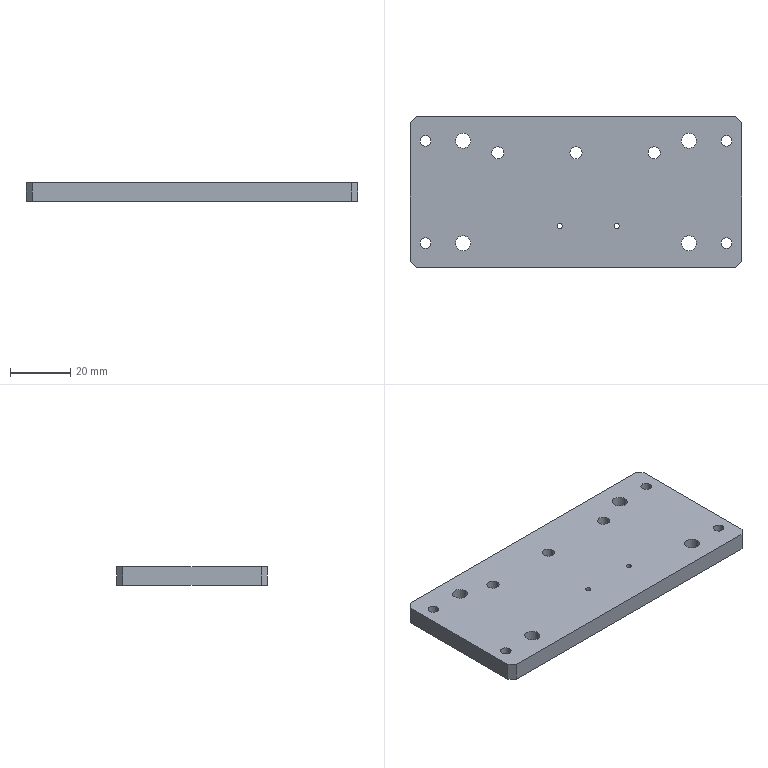Component | SolidWorks | 170423A4-SafetyPowerProbeFixingPlate1-1 | 1 solid | 48 faces | box 110 x 50 x 6 mm | volume 31593 mm3 | cylinder 34 | plane 14 | commonest cylinder face diameters 5 x8 7 x8 3.5 x8 4 x6 1.67 x4
build123d program:
from build123d import *

# Parameters (mm, degrees)
SKETCH2_W                                       = 110
SKETCH2_H                                       = 50
BOSS_EXTRUDE1_DEPTH                             = 6
F_4_0_4_DIAMETER_HOLE1_D                        = 4
M3_HEX_SOCKET_HEAD_CAP_SCREW_CBORE1_D           = 3.5
M3_HEX_SOCKET_HEAD_CAP_SCREW_CBORE1_CBORE_D     = 7
M3_HEX_SOCKET_HEAD_CAP_SCREW_CBORE1_CBORE_DEPTH = 3.5
CHAMFER1_SIZE                                   = 2
F_1_65_1_65_DIAMETER_HOLE1_D                    = 1.67
F_5_0_5_DIAMETER_HOLE1_D                        = 5


with BuildPart() as part:
    # Sketch2 → Boss-Extrude1 (new body)
    with BuildSketch(Plane.XY):
        with Locations((37.907, 35.158)):
            Rectangle(SKETCH2_W, SKETCH2_H)
    extrude(amount=BOSS_EXTRUDE1_DEPTH)

    # 4.0 _4_ Diameter Hole1 (through all)
    with Locations(Plane.XY.offset(6)):
        with Locations((11.907, 48.158), (37.907, 48.158), (63.907, 48.158)):
            Hole(F_4_0_4_DIAMETER_HOLE1_D / 2)

    # M3 Hex Socket Head Cap Screw CBORE1 (through all)
    with Locations(Plane.XY.offset(6)):
        with Locations((-12.093, 52.158), (-12.093, 18.158), (87.907, 52.158), (87.907, 18.158)):
            CounterBoreHole(M3_HEX_SOCKET_HEAD_CAP_SCREW_CBORE1_D / 2, M3_HEX_SOCKET_HEAD_CAP_SCREW_CBORE1_CBORE_D / 2, M3_HEX_SOCKET_HEAD_CAP_SCREW_CBORE1_CBORE_DEPTH)

    # Chamfer1
    chamfer1_edges = [part.edges().sort_by_distance(p)[0] for p in [
        (-17.093, 60.158, 3),
        (92.907, 60.158, 3),
        (92.907, 10.158, 3),
        (-17.093, 10.158, 3),
    ]]
    chamfer(chamfer1_edges, length=CHAMFER1_SIZE)

    # 1.65 _1.65_ Diameter Hole1 (through all)
    with Locations(Plane.XY.offset(6)):
        with Locations((24.407, 23.874), (43.359, 23.874)):
            Hole(F_1_65_1_65_DIAMETER_HOLE1_D / 2)

    # 5.0 _5_ Diameter Hole1 (through all)
    with Locations(Plane.XY.offset(6)):
        with Locations((0.4069, 52.158), (0.4069, 18.158), (75.407, 52.158), (75.407, 18.158)):
            Hole(F_5_0_5_DIAMETER_HOLE1_D / 2)


solid = part.part

# Placed as in the assembly
solid = solid.moved(Location((66.593, -20.769, -73.574), (-180, 0, 180)))